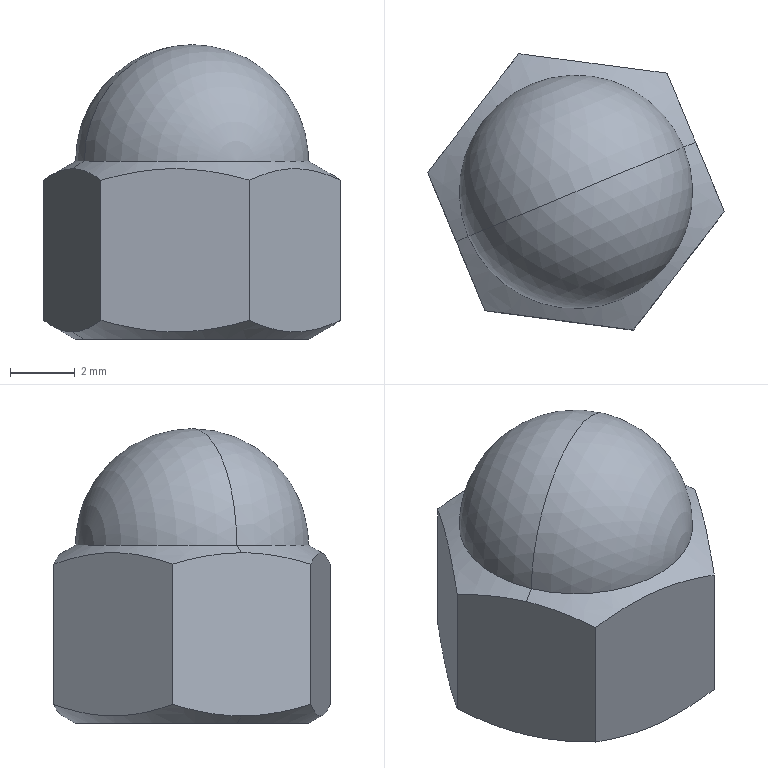Component | NX | GB_T_802_1_COMBINED_CAP_NUT_M5_5 | 1 solid | 15 faces | volume 318 mm3 | plane 8 | cone 4 | sphere 2 | cylinder 1 | commonest cylinder face diameters 5.01 x1